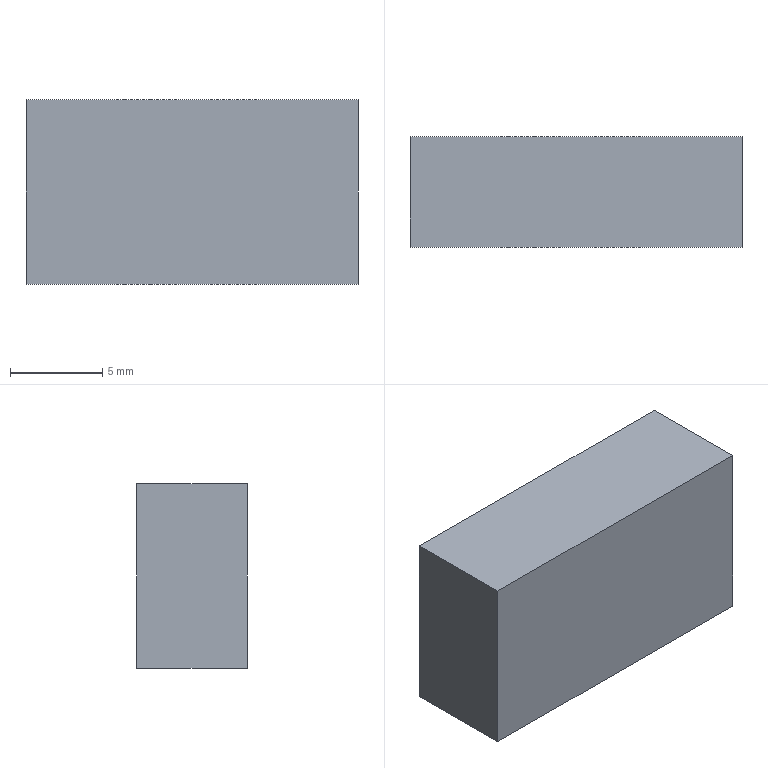Component | NX | WORKPIECE_RAW_1 | 1 solid | 6 faces | box 18 x 6 x 10 mm | volume 1080 mm3 | plane 6
STEP:
#1=CARTESIAN_POINT('',(0.,0.,0.));
#2=DIRECTION('',(0.,0.,1.));
#3=DIRECTION('',(1.,0.,0.));
#4=AXIS2_PLACEMENT_3D('',#1,#2,#3);
#5=CARTESIAN_POINT('',(-38.436,3.,6.));
#6=VERTEX_POINT('',#5);
#7=CARTESIAN_POINT('',(-56.436,3.,6.));
#8=VERTEX_POINT('',#7);
#9=CARTESIAN_POINT('',(-47.436,3.,6.));
#10=DIRECTION('',(-1.,0.,0.));
#11=VECTOR('',#10,1.);
#12=LINE('',#9,#11);
#13=CARTESIAN_POINT('',(-47.436,3.,11.));
#14=DIRECTION('',(0.,-1.,0.));
#15=DIRECTION('',(1.,0.,0.));
#16=AXIS2_PLACEMENT_3D('',#13,#14,#15);
#17=PLANE('',#16);
#18=CARTESIAN_POINT('',(0.,-5.));
#19=DIRECTION('',(-1.,0.));
#20=VECTOR('',#19,1.);
#21=LINE('',#18,#20);
#22=(GEOMETRIC_REPRESENTATION_CONTEXT(2)PARAMETRIC_REPRESENTATION_CONTEXT()REPRESENTATION_CONTEXT('',''));
#23=DEFINITIONAL_REPRESENTATION('',(#21),#22);
#24=PCURVE('',#17,#23);
#25=CARTESIAN_POINT('',(-47.436,9.,6.));
#26=DIRECTION('',(0.,0.,-1.));
#27=DIRECTION('',(0.,1.,0.));
#28=AXIS2_PLACEMENT_3D('',#25,#26,#27);
#29=PLANE('',#28);
#30=CARTESIAN_POINT('',(-6.,0.));
#31=DIRECTION('',(0.,-1.));
#32=VECTOR('',#31,1.);
#33=LINE('',#30,#32);
#34=(GEOMETRIC_REPRESENTATION_CONTEXT(2)PARAMETRIC_REPRESENTATION_CONTEXT()REPRESENTATION_CONTEXT('',''));
#35=DEFINITIONAL_REPRESENTATION('',(#33),#34);
#36=PCURVE('',#29,#35);
#37=SURFACE_CURVE('',#12,(#24,#36),.PCURVE_S1.);
#38=EDGE_CURVE('',#6,#8,#37,.T.);
#39=ORIENTED_EDGE('',*,*,#38,.F.);
#40=CARTESIAN_POINT('',(-38.436,3.,16.));
#41=VERTEX_POINT('',#40);
#42=CARTESIAN_POINT('',(-38.436,3.,11.));
#43=DIRECTION('',(0.,0.,-1.));
#44=VECTOR('',#43,1.);
#45=LINE('',#42,#44);
#46=CARTESIAN_POINT('',(9.,0.));
#47=DIRECTION('',(0.,-1.));
#48=VECTOR('',#47,1.);
#49=LINE('',#46,#48);
#50=(GEOMETRIC_REPRESENTATION_CONTEXT(2)PARAMETRIC_REPRESENTATION_CONTEXT()REPRESENTATION_CONTEXT('',''));
#51=DEFINITIONAL_REPRESENTATION('',(#49),#50);
#52=PCURVE('',#17,#51);
#53=CARTESIAN_POINT('',(-38.436,9.,11.));
#54=DIRECTION('',(1.,0.,0.));
#55=DIRECTION('',(0.,1.,0.));
#56=AXIS2_PLACEMENT_3D('',#53,#54,#55);
#57=PLANE('',#56);
#58=CARTESIAN_POINT('',(-6.,0.));
#59=DIRECTION('',(0.,-1.));
#60=VECTOR('',#59,1.);
#61=LINE('',#58,#60);
#62=(GEOMETRIC_REPRESENTATION_CONTEXT(2)PARAMETRIC_REPRESENTATION_CONTEXT()REPRESENTATION_CONTEXT('',''));
#63=DEFINITIONAL_REPRESENTATION('',(#61),#62);
#64=PCURVE('',#57,#63);
#65=SURFACE_CURVE('',#45,(#52,#64),.PCURVE_S1.);
#66=EDGE_CURVE('',#41,#6,#65,.T.);
#67=ORIENTED_EDGE('',*,*,#66,.F.);
#68=CARTESIAN_POINT('',(-56.436,3.,16.));
#69=VERTEX_POINT('',#68);
#70=CARTESIAN_POINT('',(-47.436,3.,16.));
#71=DIRECTION('',(1.,0.,0.));
#72=VECTOR('',#71,1.);
#73=LINE('',#70,#72);
#74=CARTESIAN_POINT('',(0.,5.));
#75=DIRECTION('',(1.,0.));
#76=VECTOR('',#75,1.);
#77=LINE('',#74,#76);
#78=(GEOMETRIC_REPRESENTATION_CONTEXT(2)PARAMETRIC_REPRESENTATION_CONTEXT()REPRESENTATION_CONTEXT('',''));
#79=DEFINITIONAL_REPRESENTATION('',(#77),#78);
#80=PCURVE('',#17,#79);
#81=CARTESIAN_POINT('',(-47.436,9.,16.));
#82=DIRECTION('',(0.,0.,1.));
#83=DIRECTION('',(0.,-1.,0.));
#84=AXIS2_PLACEMENT_3D('',#81,#82,#83);
#85=PLANE('',#84);
#86=CARTESIAN_POINT('',(6.,0.));
#87=DIRECTION('',(0.,1.));
#88=VECTOR('',#87,1.);
#89=LINE('',#86,#88);
#90=(GEOMETRIC_REPRESENTATION_CONTEXT(2)PARAMETRIC_REPRESENTATION_CONTEXT()REPRESENTATION_CONTEXT('',''));
#91=DEFINITIONAL_REPRESENTATION('',(#89),#90);
#92=PCURVE('',#85,#91);
#93=SURFACE_CURVE('',#73,(#80,#92),.PCURVE_S1.);
#94=EDGE_CURVE('',#69,#41,#93,.T.);
#95=ORIENTED_EDGE('',*,*,#94,.F.);
#96=CARTESIAN_POINT('',(-56.436,3.,11.));
#97=DIRECTION('',(0.,0.,1.));
#98=VECTOR('',#97,1.);
#99=LINE('',#96,#98);
#100=CARTESIAN_POINT('',(-9.,0.));
#101=DIRECTION('',(0.,1.));
#102=VECTOR('',#101,1.);
#103=LINE('',#100,#102);
#104=(GEOMETRIC_REPRESENTATION_CONTEXT(2)PARAMETRIC_REPRESENTATION_CONTEXT()REPRESENTATION_CONTEXT('',''));
#105=DEFINITIONAL_REPRESENTATION('',(#103),#104);
#106=PCURVE('',#17,#105);
#107=CARTESIAN_POINT('',(-56.436,9.,11.));
#108=DIRECTION('',(-1.,0.,0.));
#109=DIRECTION('',(0.,-1.,0.));
#110=AXIS2_PLACEMENT_3D('',#107,#108,#109);
#111=PLANE('',#110);
#112=CARTESIAN_POINT('',(6.,0.));
#113=DIRECTION('',(0.,1.));
#114=VECTOR('',#113,1.);
#115=LINE('',#112,#114);
#116=(GEOMETRIC_REPRESENTATION_CONTEXT(2)PARAMETRIC_REPRESENTATION_CONTEXT()REPRESENTATION_CONTEXT('',''));
#117=DEFINITIONAL_REPRESENTATION('',(#115),#116);
#118=PCURVE('',#111,#117);
#119=SURFACE_CURVE('',#99,(#106,#118),.PCURVE_S1.);
#120=EDGE_CURVE('',#8,#69,#119,.T.);
#121=ORIENTED_EDGE('',*,*,#120,.F.);
#122=EDGE_LOOP('',(#39,#67,#95,#121));
#123=FACE_BOUND('',#122,.T.);
#124=ADVANCED_FACE('',(#123),#17,.T.);
#125=CARTESIAN_POINT('',(-38.436,9.,6.));
#126=VERTEX_POINT('',#125);
#127=CARTESIAN_POINT('',(-38.436,9.,6.));
#128=DIRECTION('',(0.,-1.,0.));
#129=VECTOR('',#128,1.);
#130=LINE('',#127,#129);
#131=CARTESIAN_POINT('',(0.,9.));
#132=DIRECTION('',(-1.,0.));
#133=VECTOR('',#132,1.);
#134=LINE('',#131,#133);
#135=(GEOMETRIC_REPRESENTATION_CONTEXT(2)PARAMETRIC_REPRESENTATION_CONTEXT()REPRESENTATION_CONTEXT('',''));
#136=DEFINITIONAL_REPRESENTATION('',(#134),#135);
#137=PCURVE('',#29,#136);
#138=CARTESIAN_POINT('',(0.,-5.));
#139=DIRECTION('',(-1.,0.));
#140=VECTOR('',#139,1.);
#141=LINE('',#138,#140);
#142=(GEOMETRIC_REPRESENTATION_CONTEXT(2)PARAMETRIC_REPRESENTATION_CONTEXT()REPRESENTATION_CONTEXT('',''));
#143=DEFINITIONAL_REPRESENTATION('',(#141),#142);
#144=PCURVE('',#57,#143);
#145=SURFACE_CURVE('',#130,(#137,#144),.PCURVE_S1.);
#146=EDGE_CURVE('',#126,#6,#145,.T.);
#147=ORIENTED_EDGE('',*,*,#146,.T.);
#148=ORIENTED_EDGE('',*,*,#38,.T.);
#149=CARTESIAN_POINT('',(-56.436,9.,6.));
#150=VERTEX_POINT('',#149);
#151=CARTESIAN_POINT('',(-56.436,9.,6.));
#152=DIRECTION('',(0.,-1.,0.));
#153=VECTOR('',#152,1.);
#154=LINE('',#151,#153);
#155=CARTESIAN_POINT('',(0.,-9.));
#156=DIRECTION('',(-1.,0.));
#157=VECTOR('',#156,1.);
#158=LINE('',#155,#157);
#159=(GEOMETRIC_REPRESENTATION_CONTEXT(2)PARAMETRIC_REPRESENTATION_CONTEXT()REPRESENTATION_CONTEXT('',''));
#160=DEFINITIONAL_REPRESENTATION('',(#158),#159);
#161=PCURVE('',#29,#160);
#162=CARTESIAN_POINT('',(0.,-5.));
#163=DIRECTION('',(1.,0.));
#164=VECTOR('',#163,1.);
#165=LINE('',#162,#164);
#166=(GEOMETRIC_REPRESENTATION_CONTEXT(2)PARAMETRIC_REPRESENTATION_CONTEXT()REPRESENTATION_CONTEXT('',''));
#167=DEFINITIONAL_REPRESENTATION('',(#165),#166);
#168=PCURVE('',#111,#167);
#169=SURFACE_CURVE('',#154,(#161,#168),.PCURVE_S1.);
#170=EDGE_CURVE('',#150,#8,#169,.T.);
#171=ORIENTED_EDGE('',*,*,#170,.F.);
#172=CARTESIAN_POINT('',(-47.436,9.,6.));
#173=DIRECTION('',(1.,0.,0.));
#174=VECTOR('',#173,1.);
#175=LINE('',#172,#174);
#176=CARTESIAN_POINT('',(0.,0.));
#177=DIRECTION('',(0.,1.));
#178=VECTOR('',#177,1.);
#179=LINE('',#176,#178);
#180=(GEOMETRIC_REPRESENTATION_CONTEXT(2)PARAMETRIC_REPRESENTATION_CONTEXT()REPRESENTATION_CONTEXT('',''));
#181=DEFINITIONAL_REPRESENTATION('',(#179),#180);
#182=PCURVE('',#29,#181);
#183=CARTESIAN_POINT('',(-47.436,9.,11.));
#184=DIRECTION('',(0.,1.,0.));
#185=DIRECTION('',(-1.,0.,0.));
#186=AXIS2_PLACEMENT_3D('',#183,#184,#185);
#187=PLANE('',#186);
#188=CARTESIAN_POINT('',(0.,-5.));
#189=DIRECTION('',(-1.,0.));
#190=VECTOR('',#189,1.);
#191=LINE('',#188,#190);
#192=(GEOMETRIC_REPRESENTATION_CONTEXT(2)PARAMETRIC_REPRESENTATION_CONTEXT()REPRESENTATION_CONTEXT('',''));
#193=DEFINITIONAL_REPRESENTATION('',(#191),#192);
#194=PCURVE('',#187,#193);
#195=SURFACE_CURVE('',#175,(#182,#194),.PCURVE_S1.);
#196=EDGE_CURVE('',#150,#126,#195,.T.);
#197=ORIENTED_EDGE('',*,*,#196,.T.);
#198=EDGE_LOOP('',(#147,#148,#171,#197));
#199=FACE_BOUND('',#198,.T.);
#200=ADVANCED_FACE('',(#199),#29,.T.);
#201=ORIENTED_EDGE('',*,*,#170,.T.);
#202=ORIENTED_EDGE('',*,*,#120,.T.);
#203=CARTESIAN_POINT('',(-56.436,9.,16.));
#204=VERTEX_POINT('',#203);
#205=CARTESIAN_POINT('',(-56.436,9.,16.));
#206=DIRECTION('',(0.,-1.,0.));
#207=VECTOR('',#206,1.);
#208=LINE('',#205,#207);
#209=CARTESIAN_POINT('',(0.,5.));
#210=DIRECTION('',(1.,0.));
#211=VECTOR('',#210,1.);
#212=LINE('',#209,#211);
#213=(GEOMETRIC_REPRESENTATION_CONTEXT(2)PARAMETRIC_REPRESENTATION_CONTEXT()REPRESENTATION_CONTEXT('',''));
#214=DEFINITIONAL_REPRESENTATION('',(#212),#213);
#215=PCURVE('',#111,#214);
#216=CARTESIAN_POINT('',(0.,-9.));
#217=DIRECTION('',(1.,0.));
#218=VECTOR('',#217,1.);
#219=LINE('',#216,#218);
#220=(GEOMETRIC_REPRESENTATION_CONTEXT(2)PARAMETRIC_REPRESENTATION_CONTEXT()REPRESENTATION_CONTEXT('',''));
#221=DEFINITIONAL_REPRESENTATION('',(#219),#220);
#222=PCURVE('',#85,#221);
#223=SURFACE_CURVE('',#208,(#215,#222),.PCURVE_S1.);
#224=EDGE_CURVE('',#204,#69,#223,.T.);
#225=ORIENTED_EDGE('',*,*,#224,.F.);
#226=CARTESIAN_POINT('',(-56.436,9.,11.));
#227=DIRECTION('',(0.,0.,-1.));
#228=VECTOR('',#227,1.);
#229=LINE('',#226,#228);
#230=CARTESIAN_POINT('',(0.,0.));
#231=DIRECTION('',(0.,-1.));
#232=VECTOR('',#231,1.);
#233=LINE('',#230,#232);
#234=(GEOMETRIC_REPRESENTATION_CONTEXT(2)PARAMETRIC_REPRESENTATION_CONTEXT()REPRESENTATION_CONTEXT('',''));
#235=DEFINITIONAL_REPRESENTATION('',(#233),#234);
#236=PCURVE('',#111,#235);
#237=CARTESIAN_POINT('',(9.,0.));
#238=DIRECTION('',(0.,-1.));
#239=VECTOR('',#238,1.);
#240=LINE('',#237,#239);
#241=(GEOMETRIC_REPRESENTATION_CONTEXT(2)PARAMETRIC_REPRESENTATION_CONTEXT()REPRESENTATION_CONTEXT('',''));
#242=DEFINITIONAL_REPRESENTATION('',(#240),#241);
#243=PCURVE('',#187,#242);
#244=SURFACE_CURVE('',#229,(#236,#243),.PCURVE_S1.);
#245=EDGE_CURVE('',#204,#150,#244,.T.);
#246=ORIENTED_EDGE('',*,*,#245,.T.);
#247=EDGE_LOOP('',(#201,#202,#225,#246));
#248=FACE_BOUND('',#247,.T.);
#249=ADVANCED_FACE('',(#248),#111,.T.);
#250=ORIENTED_EDGE('',*,*,#224,.T.);
#251=ORIENTED_EDGE('',*,*,#94,.T.);
#252=CARTESIAN_POINT('',(-38.436,9.,16.));
#253=VERTEX_POINT('',#252);
#254=CARTESIAN_POINT('',(-38.436,9.,16.));
#255=DIRECTION('',(0.,-1.,0.));
#256=VECTOR('',#255,1.);
#257=LINE('',#254,#256);
#258=CARTESIAN_POINT('',(0.,9.));
#259=DIRECTION('',(1.,0.));
#260=VECTOR('',#259,1.);
#261=LINE('',#258,#260);
#262=(GEOMETRIC_REPRESENTATION_CONTEXT(2)PARAMETRIC_REPRESENTATION_CONTEXT()REPRESENTATION_CONTEXT('',''));
#263=DEFINITIONAL_REPRESENTATION('',(#261),#262);
#264=PCURVE('',#85,#263);
#265=CARTESIAN_POINT('',(0.,5.));
#266=DIRECTION('',(-1.,0.));
#267=VECTOR('',#266,1.);
#268=LINE('',#265,#267);
#269=(GEOMETRIC_REPRESENTATION_CONTEXT(2)PARAMETRIC_REPRESENTATION_CONTEXT()REPRESENTATION_CONTEXT('',''));
#270=DEFINITIONAL_REPRESENTATION('',(#268),#269);
#271=PCURVE('',#57,#270);
#272=SURFACE_CURVE('',#257,(#264,#271),.PCURVE_S1.);
#273=EDGE_CURVE('',#253,#41,#272,.T.);
#274=ORIENTED_EDGE('',*,*,#273,.F.);
#275=CARTESIAN_POINT('',(-47.436,9.,16.));
#276=DIRECTION('',(-1.,0.,0.));
#277=VECTOR('',#276,1.);
#278=LINE('',#275,#277);
#279=CARTESIAN_POINT('',(0.,0.));
#280=DIRECTION('',(0.,-1.));
#281=VECTOR('',#280,1.);
#282=LINE('',#279,#281);
#283=(GEOMETRIC_REPRESENTATION_CONTEXT(2)PARAMETRIC_REPRESENTATION_CONTEXT()REPRESENTATION_CONTEXT('',''));
#284=DEFINITIONAL_REPRESENTATION('',(#282),#283);
#285=PCURVE('',#85,#284);
#286=CARTESIAN_POINT('',(0.,5.));
#287=DIRECTION('',(1.,0.));
#288=VECTOR('',#287,1.);
#289=LINE('',#286,#288);
#290=(GEOMETRIC_REPRESENTATION_CONTEXT(2)PARAMETRIC_REPRESENTATION_CONTEXT()REPRESENTATION_CONTEXT('',''));
#291=DEFINITIONAL_REPRESENTATION('',(#289),#290);
#292=PCURVE('',#187,#291);
#293=SURFACE_CURVE('',#278,(#285,#292),.PCURVE_S1.);
#294=EDGE_CURVE('',#253,#204,#293,.T.);
#295=ORIENTED_EDGE('',*,*,#294,.T.);
#296=EDGE_LOOP('',(#250,#251,#274,#295));
#297=FACE_BOUND('',#296,.T.);
#298=ADVANCED_FACE('',(#297),#85,.T.);
#299=CARTESIAN_POINT('',(-38.436,9.,11.));
#300=DIRECTION('',(0.,0.,1.));
#301=VECTOR('',#300,1.);
#302=LINE('',#299,#301);
#303=CARTESIAN_POINT('',(-9.,0.));
#304=DIRECTION('',(0.,1.));
#305=VECTOR('',#304,1.);
#306=LINE('',#303,#305);
#307=(GEOMETRIC_REPRESENTATION_CONTEXT(2)PARAMETRIC_REPRESENTATION_CONTEXT()REPRESENTATION_CONTEXT('',''));
#308=DEFINITIONAL_REPRESENTATION('',(#306),#307);
#309=PCURVE('',#187,#308);
#310=CARTESIAN_POINT('',(0.,0.));
#311=DIRECTION('',(0.,1.));
#312=VECTOR('',#311,1.);
#313=LINE('',#310,#312);
#314=(GEOMETRIC_REPRESENTATION_CONTEXT(2)PARAMETRIC_REPRESENTATION_CONTEXT()REPRESENTATION_CONTEXT('',''));
#315=DEFINITIONAL_REPRESENTATION('',(#313),#314);
#316=PCURVE('',#57,#315);
#317=SURFACE_CURVE('',#302,(#309,#316),.PCURVE_S1.);
#318=EDGE_CURVE('',#126,#253,#317,.T.);
#319=ORIENTED_EDGE('',*,*,#318,.F.);
#320=ORIENTED_EDGE('',*,*,#196,.F.);
#321=ORIENTED_EDGE('',*,*,#245,.F.);
#322=ORIENTED_EDGE('',*,*,#294,.F.);
#323=EDGE_LOOP('',(#319,#320,#321,#322));
#324=FACE_BOUND('',#323,.T.);
#325=ADVANCED_FACE('',(#324),#187,.T.);
#326=ORIENTED_EDGE('',*,*,#318,.T.);
#327=ORIENTED_EDGE('',*,*,#273,.T.);
#328=ORIENTED_EDGE('',*,*,#66,.T.);
#329=ORIENTED_EDGE('',*,*,#146,.F.);
#330=EDGE_LOOP('',(#326,#327,#328,#329));
#331=FACE_BOUND('',#330,.T.);
#332=ADVANCED_FACE('',(#331),#57,.T.);
#333=CLOSED_SHELL('',(#124,#200,#249,#298,#325,#332));
#334=MANIFOLD_SOLID_BREP('',#333);
#335=(LENGTH_UNIT()NAMED_UNIT(*)SI_UNIT(.MILLI.,.METRE.));
#336=UNCERTAINTY_MEASURE_WITH_UNIT(LENGTH_MEASURE(0.0000001),#335,'','');
#337=(NAMED_UNIT(*)PLANE_ANGLE_UNIT()SI_UNIT($,.RADIAN.));
#338=(NAMED_UNIT(*)SI_UNIT($,.STERADIAN.)SOLID_ANGLE_UNIT());
#339=(GEOMETRIC_REPRESENTATION_CONTEXT(3)GLOBAL_UNCERTAINTY_ASSIGNED_CONTEXT((#336))GLOBAL_UNIT_ASSIGNED_CONTEXT((#335,#337,#338))REPRESENTATION_CONTEXT('',''));
#340=ADVANCED_BREP_SHAPE_REPRESENTATION('',(#4,#334),#339);